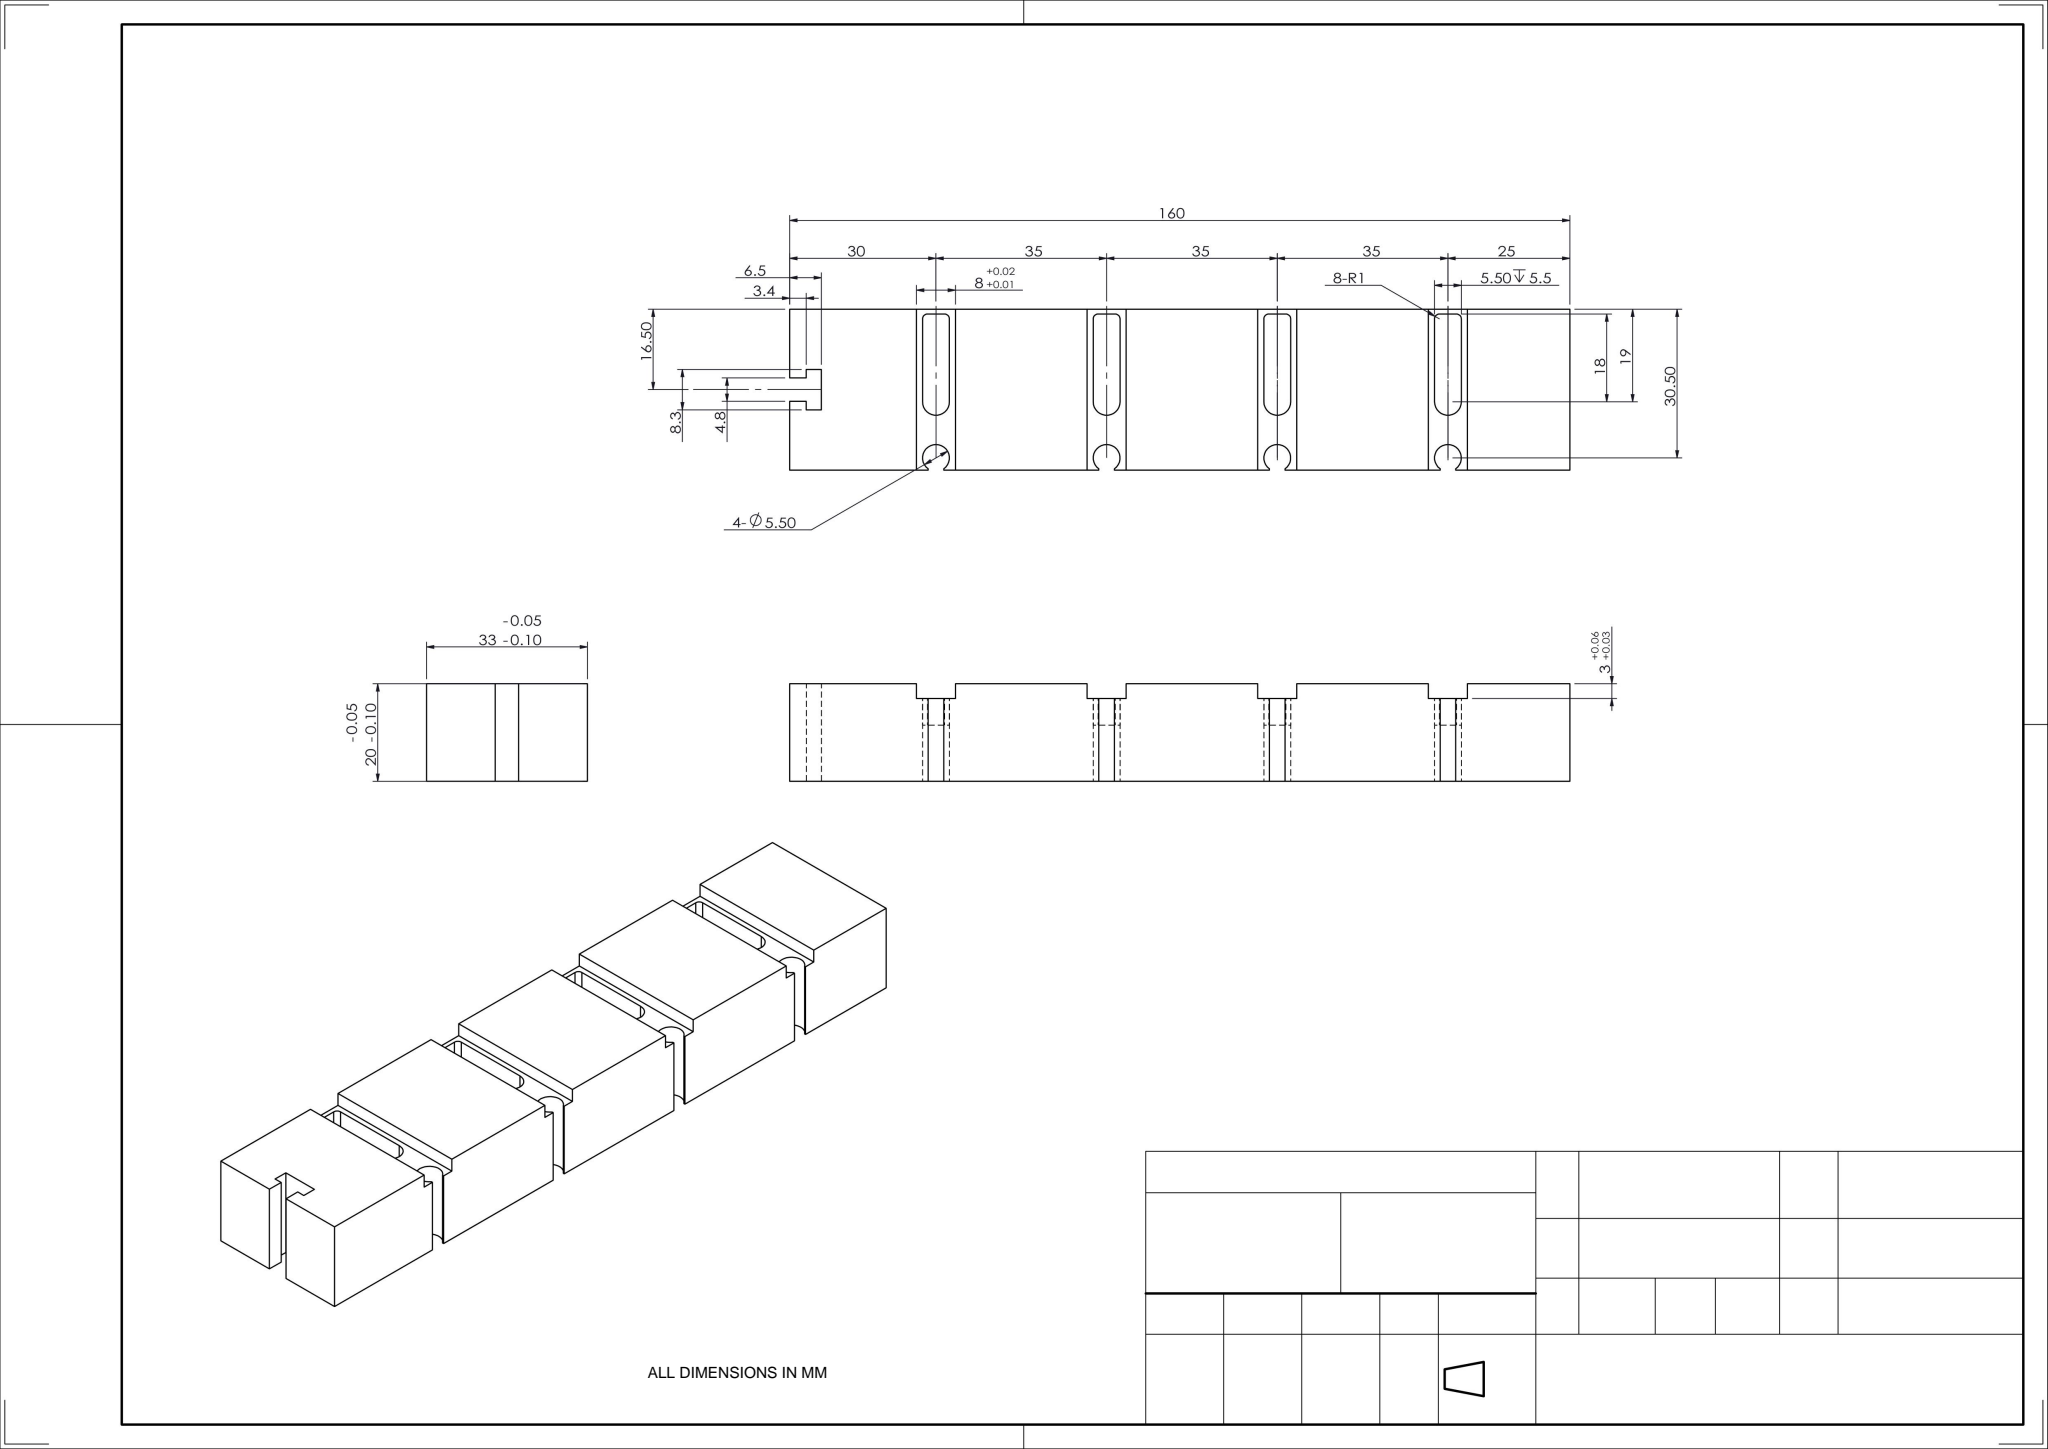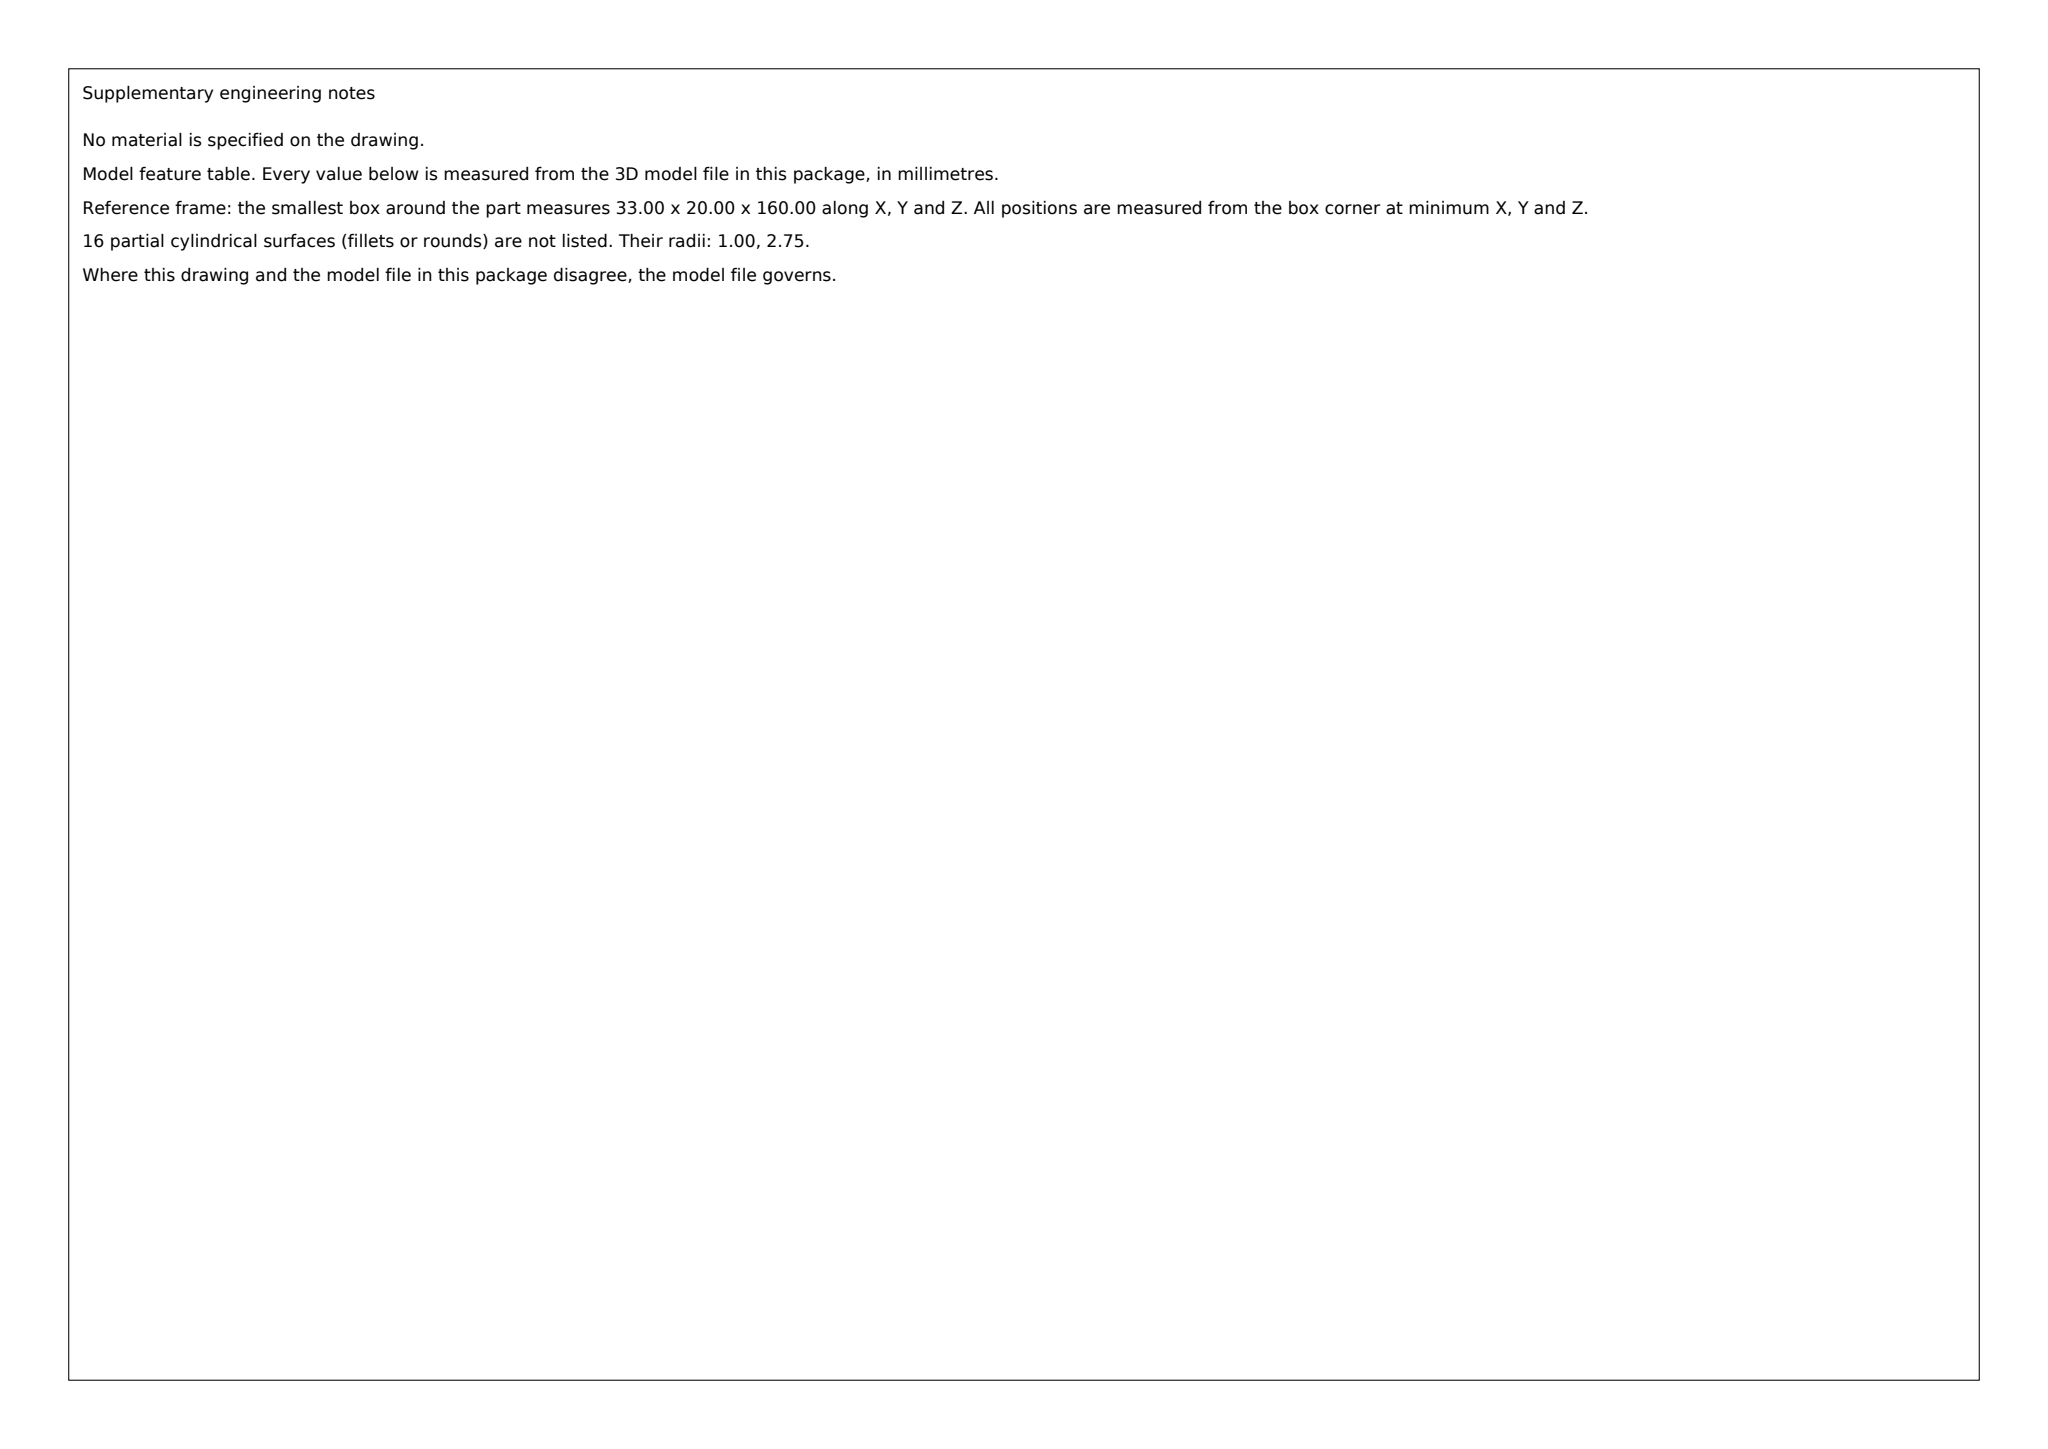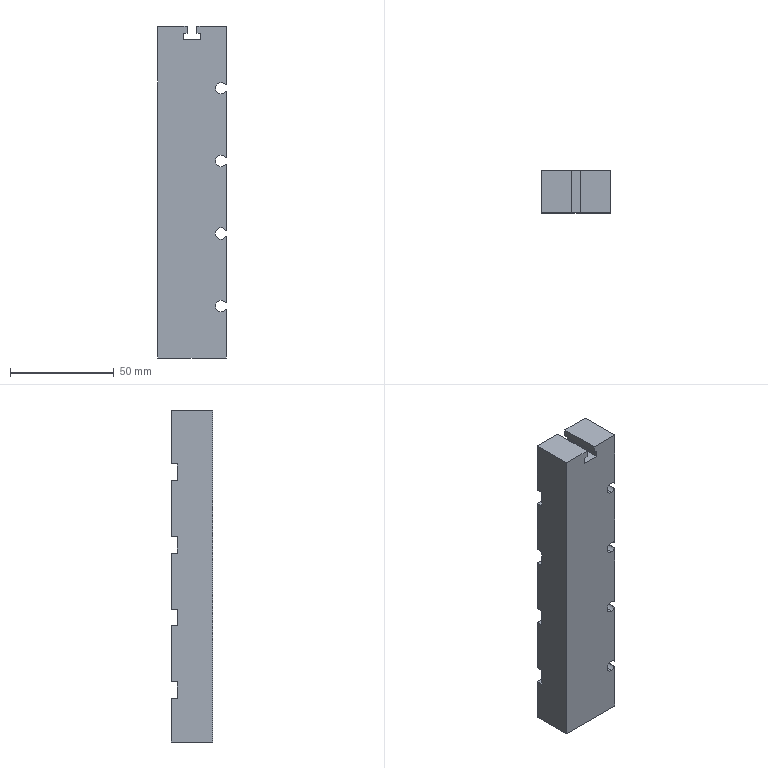Part | SolidWorks | mm | 1 solid | 82 faces | box 33 x 20 x 160 mm | volume 97564 mm3 | plane 58 | cylinder 24 | commonest cylinder face diameters 5.5 x16 2 x8
build123d program:
from build123d import *

# Parameters (mm, degrees)
SKETCH1_W                      = 33
SKETCH1_H                      = 20
EXTRUDE1_DEPTH                 = 160
SKETCH2_W                      = 33
SKETCH2_H                      = 8
CUT_EXTRUDE1_DEPTH             = 3
CUT_EXTRUDE2_REACH             = 177.477
CUT_EXTRUDE2_DIRECTION_2_DEPTH = 10
LPATTERN1_COUNT                = 4
LPATTERN1_PITCH                = 35
CUT_EXTRUDE3_REACH             = 177.793
CUT_EXTRUDE4_DEPTH             = 5.5
LPATTERN2_COUNT                = 4
LPATTERN2_PITCH                = 35


with BuildPart() as part:
    # Sketch1 → Extrude1 (new body)
    with BuildSketch(Plane.XY):
        with Locations((-53.523, 24.506)):
            Rectangle(SKETCH1_W, SKETCH1_H)
    extrude(amount=EXTRUDE1_DEPTH)

    # Sketch2 → Cut-Extrude1 (cut)
    with BuildSketch(Plane(origin=(0, 34.506, 0), x_dir=(1, 0, 0), z_dir=(0, 1, 0))):
        with Locations((-53.523, -130)):
            Rectangle(SKETCH2_W, SKETCH2_H)
    cut_extrude1 = extrude(amount=-CUT_EXTRUDE1_DEPTH, mode=Mode.SUBTRACT)

    # Sketch3 → Cut-Extrude2 (cut, up to next)
    with BuildSketch(Plane(origin=(0, 31.506, 0), x_dir=(1, 0, 0), z_dir=(0, 1, 0)), mode=Mode.PRIVATE) as cut_extrude2_sk1:
        with BuildLine():
            Line((-37.023, -128.4), (-37.023, -131.6))
            Line((-37.023, -131.6), (-37.286, -131.6))
            ThreePointArc((-37.286, -131.6), (-42.273, -130), (-37.286, -128.4))
            Line((-37.286, -128.4), (-37.023, -128.4))
        make_face()
    cut_extrude2_tool1 = extrude(cut_extrude2_sk1.sketch, amount=-CUT_EXTRUDE2_REACH, mode=Mode.PRIVATE) & part.part
    cut_extrude2 = cut_extrude2_tool1.solids().sort_by_distance((-39.554, 31.506, 130))[0]
    add(cut_extrude2, mode=Mode.SUBTRACT)

    # Sketch3 → Cut-Extrude2 direction 2 (cut)
    with BuildSketch(Plane(origin=(0, 31.506, 0), x_dir=(1, 0, 0), z_dir=(0, 1, 0))):
        with BuildLine():
            Line((-37.023, -128.4), (-37.023, -131.6))
            Line((-37.023, -131.6), (-37.286, -131.6))
            ThreePointArc((-37.286, -131.6), (-42.273, -130), (-37.286, -128.4))
            Line((-37.286, -128.4), (-37.023, -128.4))
        make_face()
    cut_extrude2_direction_2 = extrude(amount=CUT_EXTRUDE2_DIRECTION_2_DEPTH, mode=Mode.SUBTRACT)

    # LPattern1: Cut-Extrude1, Cut-Extrude2, Cut-Extrude2 direction 2 ×4
    with Locations(*[(0, 0, -i * LPATTERN1_PITCH) for i in range(1, LPATTERN1_COUNT)]):
        add(cut_extrude1, mode=Mode.SUBTRACT)
        add(cut_extrude2, mode=Mode.SUBTRACT)
        add(cut_extrude2_direction_2, mode=Mode.SUBTRACT)

    # Sketch4 → Cut-Extrude3 (cut, up to next)
    with BuildSketch(Plane(origin=(0, 34.506, 0), x_dir=(1, 0, 0), z_dir=(0, 1, 0)), mode=Mode.PRIVATE) as cut_extrude3_sk1:
        Polygon((-55.923, -160), (-55.923, -156.6), (-57.673, -156.6), (-57.673, -153.5), (-49.373, -153.5), (-49.373, -156.6), (-51.123, -156.6), (-51.123, -160), align=None)
    cut_extrude3_tool1 = extrude(cut_extrude3_sk1.sketch, amount=-CUT_EXTRUDE3_REACH, mode=Mode.PRIVATE) & part.part
    add(cut_extrude3_tool1.solids().sort_by_distance((-53.523, 34.506, 156.311))[0], mode=Mode.SUBTRACT)

    # Sketch5 → Cut-Extrude4 (cut)
    with BuildSketch(Plane(origin=(0, 31.506, 0), x_dir=(-1, 0, 0), z_dir=(0, 1, 0))):
        with BuildLine():
            Line((51.023, 127.25), (68.023, 127.25))
            ThreePointArc((68.023, 127.25), (68.73, 127.543), (69.023, 128.25))
            Line((69.023, 128.25), (69.023, 131.75))
            ThreePointArc((69.023, 131.75), (68.73, 132.457), (68.023, 132.75))
            Line((68.023, 132.75), (51.023, 132.75))
            ThreePointArc((51.023, 132.75), (48.273, 130), (51.023, 127.25))
        make_face()
    cut_extrude4 = extrude(amount=-CUT_EXTRUDE4_DEPTH, mode=Mode.SUBTRACT)

    # LPattern2: Cut-Extrude4 ×4
    with Locations(*[(0, 0, -i * LPATTERN2_PITCH) for i in range(1, LPATTERN2_COUNT)]):
        add(cut_extrude4, mode=Mode.SUBTRACT)


solid = part.part